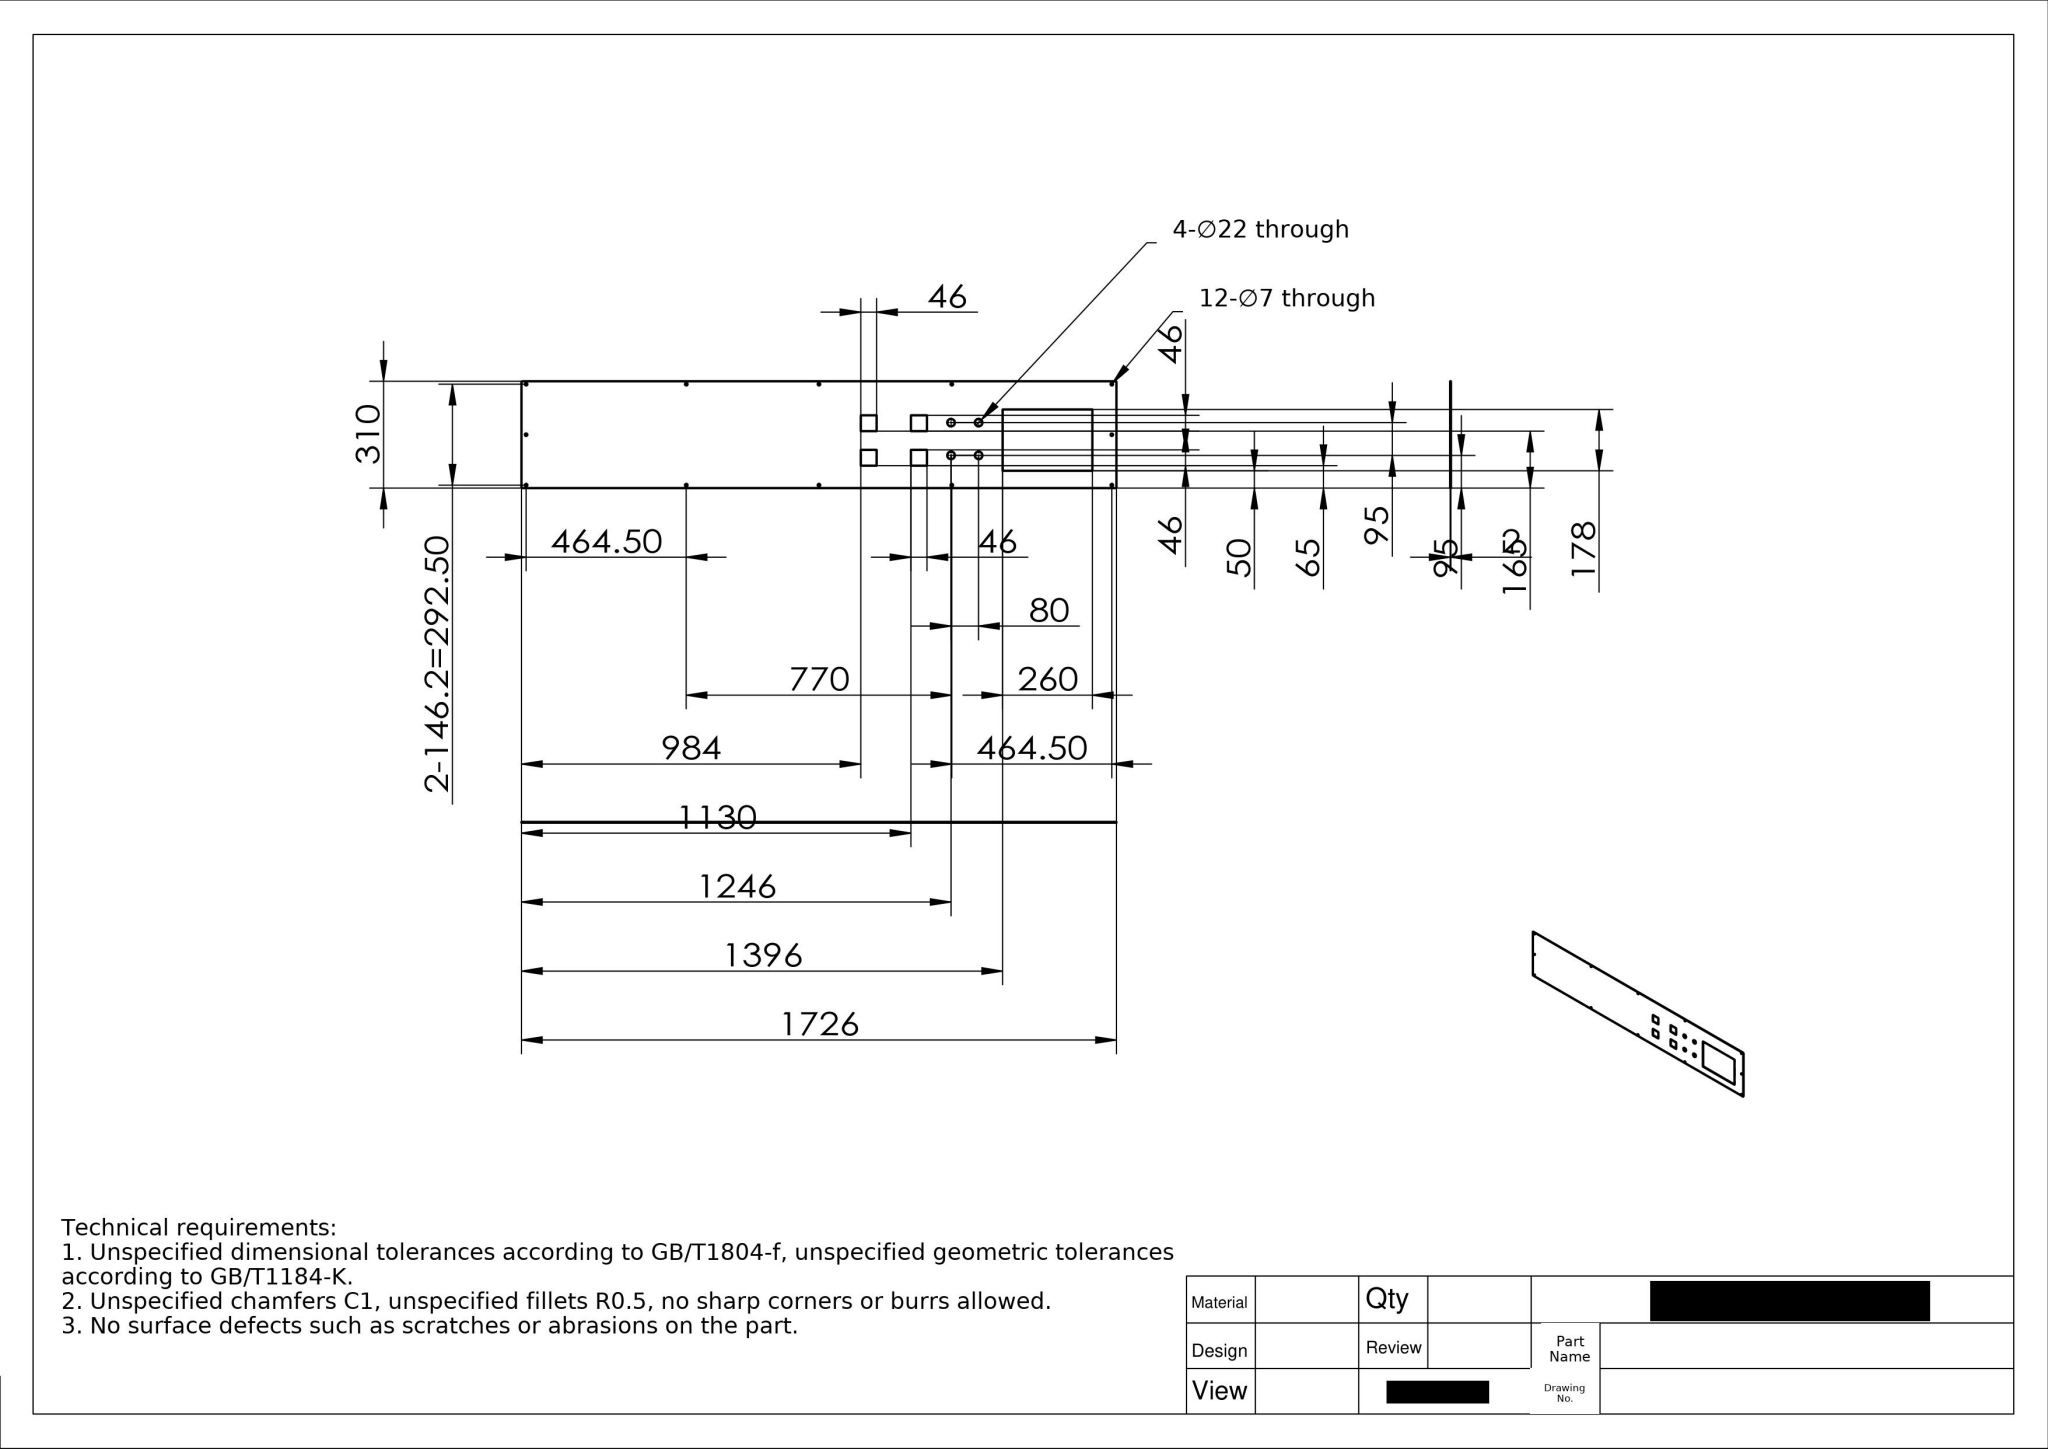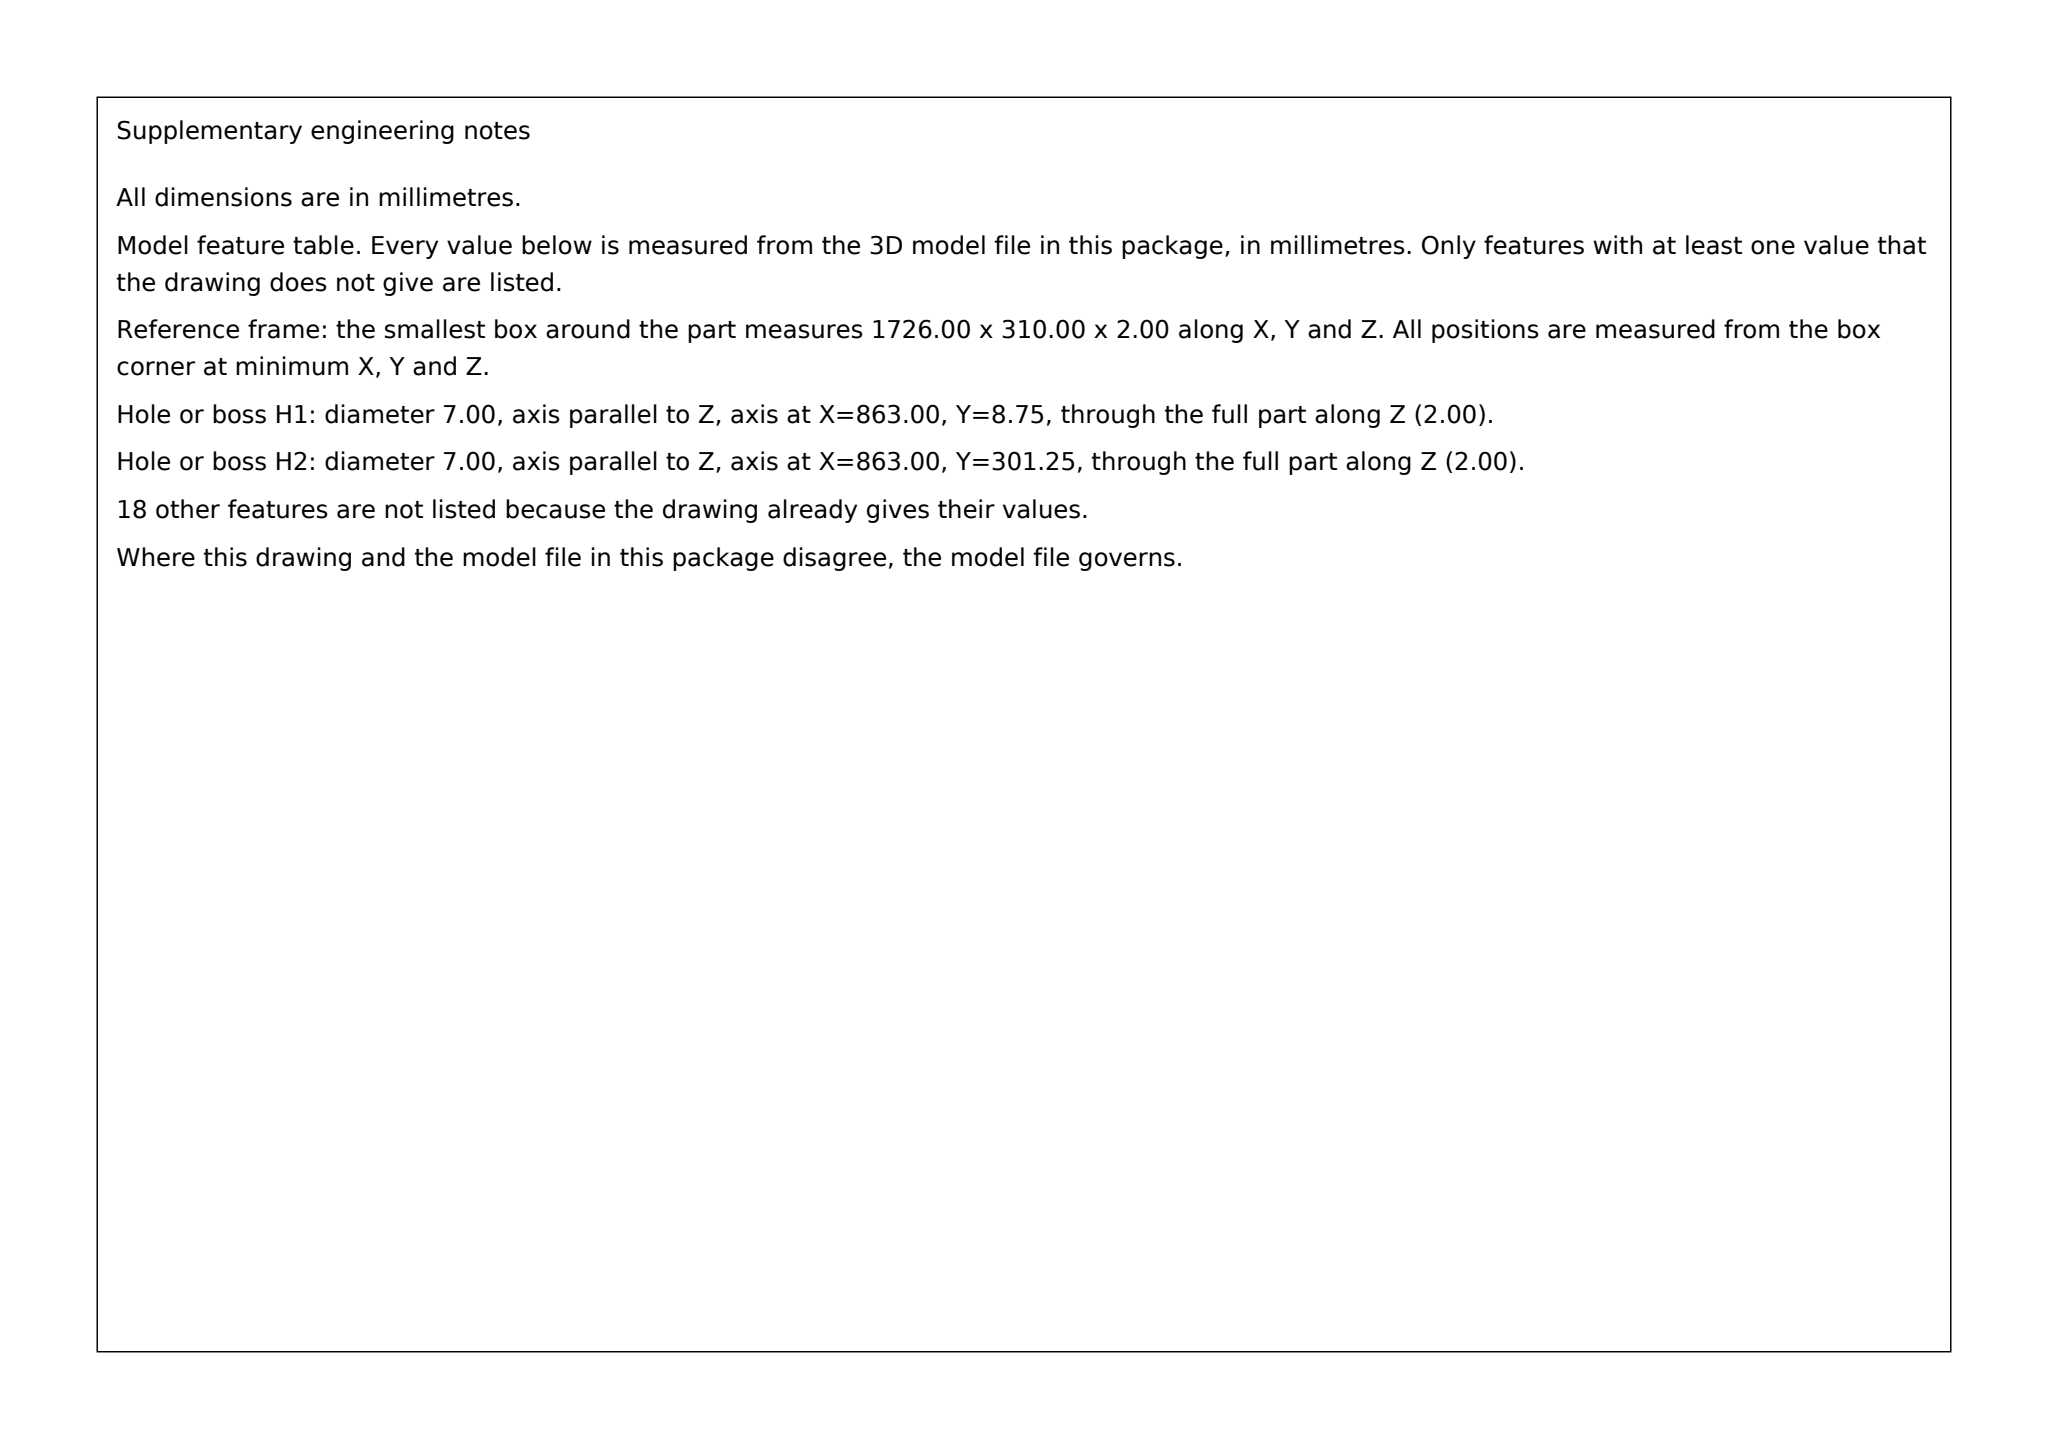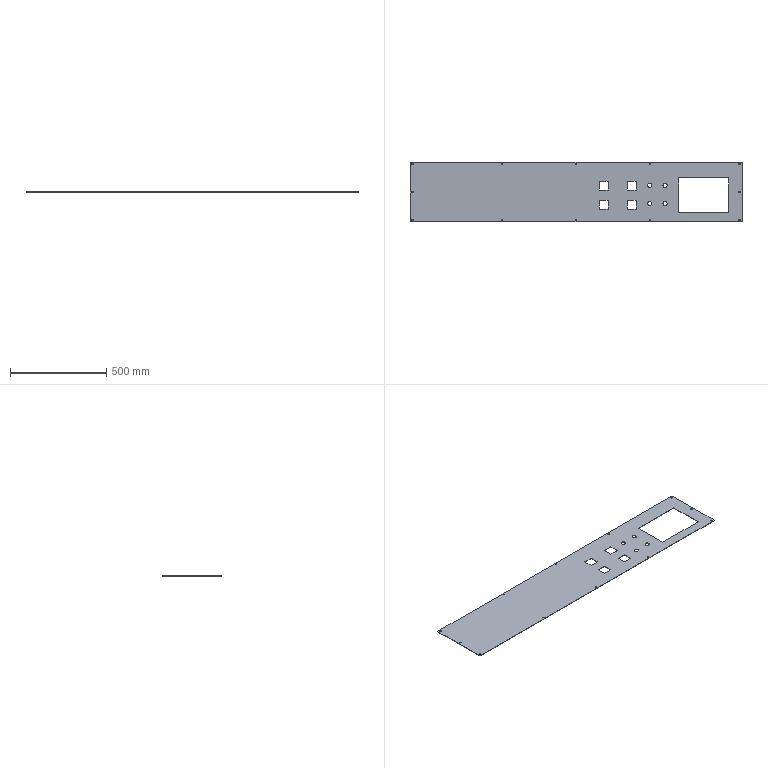Part | SolidWorks | mm | 1 solid | 62 faces | box 1726 x 310 x 2 mm | volume 956652 mm3 | cylinder 36 | plane 26 | commonest cylinder face diameters 7 x24 22 x8 6 x4
build123d program:
from build123d import *

# Parameters (mm, degrees)
SKETCH1_W           = 1726
SKETCH1_H           = 310
BOSS_EXTRUDE1_DEPTH = 2
FILLET1_R           = 3
SKETCH2_W           = 260
SKETCH2_H           = 178
CUT_EXTRUDE1_DEPTH  = 1754.619
SKETCH3_R           = 11
CUT_EXTRUDE2_DEPTH  = 1754.619
SKETCH4_R           = 3.5
CUT_EXTRUDE3_DEPTH  = 10
SKETCH5_W           = 46
SKETCH5_H           = 46
CUT_EXTRUDE4_DEPTH  = 10
LPATTERN1_COUNT     = 2
LPATTERN1_PITCH     = 80
LPATTERN2_COUNT     = 2
LPATTERN2_PITCH     = 100


with BuildPart() as part:
    # Sketch1 → Boss-Extrude1 (new body)
    with BuildSketch(Plane.XY):
        with Locations((863, 155)):
            Rectangle(SKETCH1_W, SKETCH1_H)
    extrude(amount=BOSS_EXTRUDE1_DEPTH)

    # Fillet1
    fillet1_edges = [part.edges().sort_by_distance(p)[0] for p in [
        (0, 310, 1),
        (1726, 310, 1),
        (1726, 0, 1),
        (0, 0, 1),
    ]]
    fillet(fillet1_edges, radius=FILLET1_R)

    # Sketch2 → Cut-Extrude1 (cut, through all)
    with BuildSketch(Plane.XY.offset(2)):
        with Locations((1526, 139)):
            Rectangle(SKETCH2_W, SKETCH2_H)
    extrude(amount=-CUT_EXTRUDE1_DEPTH, mode=Mode.SUBTRACT)

    # Sketch3 → Cut-Extrude2 (cut, through all)
    with BuildSketch(Plane(origin=(0, 0, 0), x_dir=(-1, 0, 0), z_dir=(0, 0, -1))):
        with Locations((-1326, 95)):
            Circle(SKETCH3_R)
        with Locations((-1326, 190)):
            Circle(SKETCH3_R)
    cut_extrude2 = extrude(amount=-CUT_EXTRUDE2_DEPTH, mode=Mode.SUBTRACT)

    # Sketch4 → Cut-Extrude3 (cut)
    with BuildSketch(Plane(origin=(0, 0, 0), x_dir=(-1, 0, 0), z_dir=(0, 0, -1))):
        with Locations((-1712.5, 301.25)):
            Circle(SKETCH4_R)
        with Locations((-1712.5, 8.75)):
            Circle(SKETCH4_R)
        with Locations((-13.5, 301.25)):
            Circle(SKETCH4_R)
        with Locations((-13.5, 8.75)):
            Circle(SKETCH4_R)
        with Locations((-1248, 301.25)):
            Circle(SKETCH4_R)
        with Locations((-478, 301.25)):
            Circle(SKETCH4_R)
        with Locations((-478, 8.75)):
            Circle(SKETCH4_R)
        with Locations((-1248, 8.75)):
            Circle(SKETCH4_R)
        with Locations((-1712.5, 155)):
            Circle(SKETCH4_R)
        with Locations((-13.5, 155)):
            Circle(SKETCH4_R)
        with Locations((-863, 8.75)):
            Circle(SKETCH4_R)
        with Locations((-863, 301.25)):
            Circle(SKETCH4_R)
    extrude(amount=-CUT_EXTRUDE3_DEPTH, mode=Mode.SUBTRACT)

    # Sketch5 → Cut-Extrude4 (cut)
    with BuildSketch(Plane(origin=(0, 0, 0), x_dir=(-1, 0, 0), z_dir=(0, 0, -1))):
        with Locations((-1007, 88)):
            Rectangle(SKETCH5_W, SKETCH5_H)
        with Locations((-1153, 88)):
            Rectangle(SKETCH5_W, SKETCH5_H)
    cut_extrude4 = extrude(amount=-CUT_EXTRUDE4_DEPTH, mode=Mode.SUBTRACT)

    # LPattern1: Cut-Extrude2 ×2
    with Locations(*[(-i * LPATTERN1_PITCH, 0, 0) for i in range(1, LPATTERN1_COUNT)]):
        add(cut_extrude2, mode=Mode.SUBTRACT)

    # LPattern2: Cut-Extrude4 ×2
    with Locations(*[(0, i * LPATTERN2_PITCH, 0) for i in range(1, LPATTERN2_COUNT)]):
        add(cut_extrude4, mode=Mode.SUBTRACT)


solid = part.part